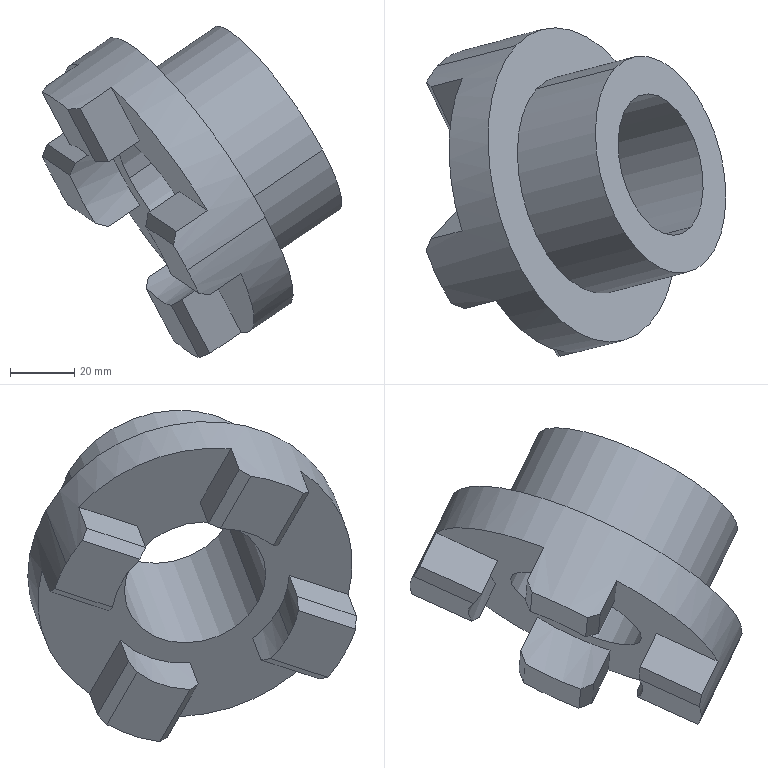Component | SolidWorks | MotorCrusherFrameCoupling-1 | 1 solid | 34 faces | volume 188214 mm3 | plane 23 | cylinder 11 | commonest cylinder face diameters 60 x5 69 x2 45 x2 100 x2